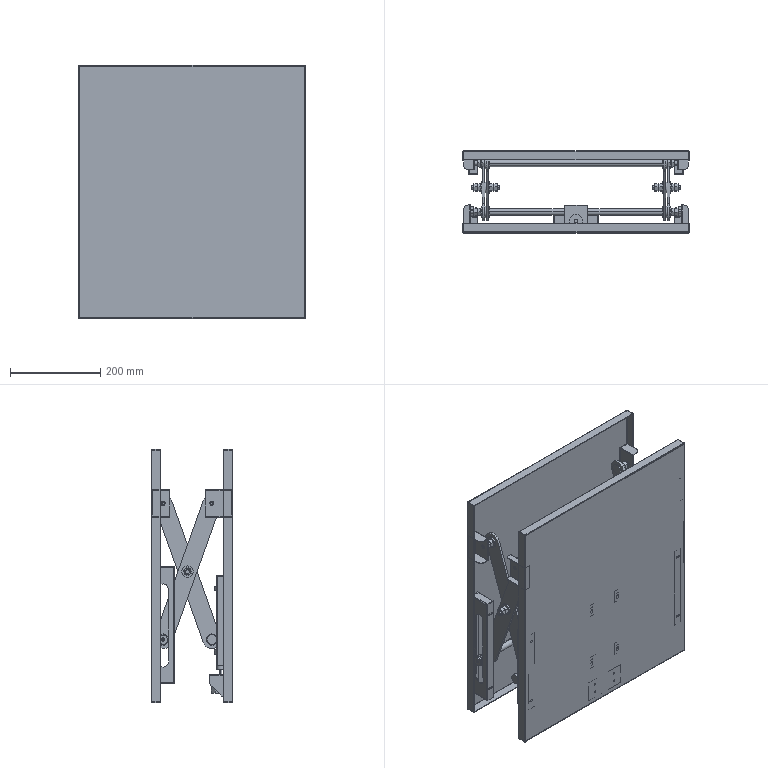Assembly | SolidWorks | mm | 92 component files | 92 solids | 1755 faces | box 500 x 180.82 x 560 mm | volume 1786102 mm3 | plane 890 | cylinder 649 | cone 208 | torus 8 | commonest cylinder face diameters 5 x77 9 x72 0.2 x51 10 x50 19 x48 4 x40 11 x32 25 x32
Bill of materials:
42StepperMotor | 1 |  | Prismatic block, square in plan with chamfered vertical corners (octagonal outline), with a short circular boss and a slender cylindrical shaft rising from the centre of one end face; small holes sit near the corners of the end face.
6800Bearing10-19-5 | 12 |  | Thick annular ring (washer- or spacer-like) with a large central through bore; axial thickness is fairly large compared with the radial wall.
Baffle | 16 |  | Flat annular washer-like disc with a central through hole; thinner than the ring part and with a smaller bore relative to its outer diameter.
Baffle2 | 2 |  | Thin flat disc with a small central through hole (fender-washer-like proportions: large outer diameter relative to the hole).
BearingHousing | 2 |  | Lug or bracket of constant-thickness profile: a rectangular base bar with a rounded (arched) tab rising from its centre. The tab has a through hole on the arch axis, and the base bar has two through holes running perpendicular to the tab hole.
BearingHousingBracket | 2 |  | Sheet-metal hat-section bracket: a central U-shaped channel with an outward flat flange on each side. Each flange has an elongated slot, and the channel web has two small round holes that appear to have slightly raised or formed rims.
AxisFixingPlate | 2 |  | Sheet-metal U/C-channel: a flat rectangular web with two parallel flanges whose free ends are rounded, and a single off-centre round through hole in the web.
BottomPlate | 1 |  | Thin flat rectangular plate, nearly square, with no visible holes or cutouts.
ConnectingRod1 | 4 |  | Thin flat link bar with fully rounded ends and three round through holes: one near each end and one at the midpoint.
Coupling2 | 1 |  | Cylindrical tube or spacer with a concentric through bore; its length is longer than its outer diameter.
FixedRotatingShaft | 4 |  | Flanged, stepped cylindrical pin or bushing: a thin large-diameter disc head, then a short larger-diameter shank section, then a longer slightly smaller-diameter shank. There is an axial bore at the free (small) end.
GuideRail | 2 |  | Elongated sheet-metal folded channel or cover strip of rectangular box-like section. One narrow face has two oblong slots near its ends, and the folded edges show rounded bend corners.
GuideRail2 | 2 |  | Tall, narrow U-shaped channel that looks like bent thin sheet. The web has one long slot that ends in a larger circular opening, like a keyhole. Each side flange has two small slotted holes, one near each end.
hex nuts, style 1-grades ab gb | 24 |  | Hexagonal nut shape with a round hole through the centre and chamfered corners on both faces.
JS60822-7C1L8M6ExternalThreadBearing | 2 |  | Turned stepped pin: a large disc-shaped head, a short collar of middle diameter, and a smaller cylindrical shank.
MotorFixture | 1 |  | Bent bracket that looks like sheet metal, with three faces. The top plate has a large central hole with four small holes in a square around it. One side flange has four holes in a rectangle. The end flange has an angled cut and a rounded corner.
PushRod | 1 |  | Long, slender stepped shaft. The main body is round, and each end steps down twice to a smaller journal. There are two ring-shaped lines near the middle of the body.
PushRod3 | 1 |  | Long, slender stepped shaft like part-63ce, but with a plain main body. Each end steps down twice to smaller diameters.
RotatingShaft | 2 |  | Turned pin with a thin round flange in the middle. A short hub of larger diameter sits on each side of the flange, and a long plain cylindrical section runs out from each hub.
ShaftRetainingRing-15 | 2 |  | Flat, open C-shaped ring with a rectangular cross-section and one gap cut straight through the ring wall.
Slider | 1 |  | Solid rectangular block. The top face has a round through-hole set off-centre, with four smaller holes in a square around it. One end face has a larger round hole set off-centre.
T8LeadScrew | 1 |  | Plain solid cylindrical rod with flat ends.
TLeadScrewNut | 1 |  | Flanged bushing: a round flange with four through-holes, a tube-shaped boss with a central through-bore on one side, and a short spigot on the other side.
AxisFixingPlate2 | 2 |  | U-shaped channel bracket that looks like bent sheet. The back web has one round hole, and the two parallel flanges have one rounded corner each.
TopPlate | 1 |  | Thin flat rectangular plate, close to square (somewhat taller than wide in the face view), with uniform thickness and plain flat faces.
U8-24-11SlotWidth6SlotDepth2 | 2 |  | Round wheel or disc shaped like a pulley, with a central through bore and a concave, rounded (roughly semicircular) groove around its outer edge between two flat-sided flanges.
Mates:
1. coincident | 42StepperMotor-1 face at (0, 0, 0) dir (0, 0, 1) | assembly plane at (0, 0, 0) dir (0, 0, 1)
2. coincident | 42StepperMotor-1 plane at (0, 0, -39) dir (0, 1, 0) | assembly plane at (0, 0, 0) dir (0, 1, 0)
3. coincident | 42StepperMotor-1 plane at (0, 0, -39) dir (1, 0, 0) | assembly plane at (0, 0, 0) dir (1, 0, 0)
4. concentric | 42StepperMotor-1 face at (0, 0, 2) dir (0, 0, -1) r 11 | MotorFixture-1 face at (0, 0, -33.941) dir (0, 0, 1) r 12
5. coincident | 42StepperMotor-1 face at (0, 0, 0) dir (0, 0, 1) | MotorFixture-1 face at (0, -25, 0) dir (0, 0, -1)
6. parallel | 42StepperMotor-1 face at (-21, 21, 0) dir (0, 1, 0) | MotorFixture-1 face at (0, -25, 1.5) dir (0, -1, 0)
7. concentric | 42StepperMotor-1 face at (0, 0, 22.5) dir (0, 0, -1) r 2.5 | Coupling2-1 face at (0, 0, 6.5) dir (0, 0, 1) r 2.5
8. coincident | 42StepperMotor-1 face at (0, 0, 22.5) dir (0, 0, 1) | Coupling2-1 face at (0, 0, 22.5) dir (0, 0, 1)
9. coincident | Coupling2-1 plane at (0, 0, 26) dir (0, -1, 0) | assembly plane at (0, 0, 0) dir (0, 1, 0)
10. concentric | Coupling2-1 face at (0, 0, 22.5) dir (0, 0, 1) r 4 | T8LeadScrew-1 face at (0, 0, 202.5) dir (0, 0, -1) r 4
11. coincident | Coupling2-1 face at (0, 0, 22.5) dir (0, 0, 1) | T8LeadScrew-1 face at (0, 0, 22.5) dir (0, 0, -1)
12. parallel | 42StepperMotor-1 face at (-21, 21, 0) dir (0, 1, 0) | T8LeadScrew-1 plane at (0, 0, 112.5) dir (0, -1, 0)
13. concentric | T8LeadScrew-1 face at (0, 0, 202.5) dir (0, 0, -1) r 4 | BearingHousing-1 face at (0, 0, 56.5) dir (0, 0, -1) r 4
14. parallel | 42StepperMotor-1 face at (-21, 21, 0) dir (0, 1, 0) | BearingHousing-1 face at (14.5, -10, 56.5) dir (0, 1, 0)
15. concentric | T8LeadScrew-1 face at (0, 0, 202.5) dir (0, 0, -1) r 4 | TLeadScrewNut-1 face at (0, 0, 63.712) dir (0, 0, -1) r 4
16. concentric | TLeadScrewNut-1 face at (0, 0, 63.712) dir (0, 0, -1) r 5 | Slider-1 face at (0, 0, 54.787) dir (0, 0, 1) r 5.1
17. coincident | TLeadScrewNut-1 face at (0, 0, 69.212) dir (0, 0, 1) | Slider-1 face at (0, 12.5, 69.212) dir (0, 0, -1)
18. concentric | Slider-1 face at (46.496, 20, 79.212) dir (-1, 0, 0) r 7.6 | PushRod-1 face at (191, 20, 79.212) dir (-1, 0, 0) r 7.5
19. width | PushRod-1 face at (191, 20, 79.212) dir (1, 0, 0) | PushRod-1 face at (-191, 20, 79.212) dir (-1, 0, 0) | Slider-1 face at (-25, 35, 69.212) dir (-1, 0, 0) | Slider-1 face at (25, 35, 69.212) dir (1, 0, 0)
20. parallel | Slider-1 face at (0, 12.5, 69.212) dir (0, 0, -1) | PushRod-1 plane at (0, 20, 79.212) dir (0, 0, 1)
21. concentric | T8LeadScrew-1 face at (0, 0, 202.5) dir (0, 0, -1) r 4 | BearingHousing-2 face at (0, 0, 197.5) dir (0, 0, -1) r 4
22. distance | BearingHousing-2 face at (0, 0, 197.5) dir (0, 0, 1) | T8LeadScrew-1 face at (0, 0, 202.5) dir (0, 0, 1)
23. coincident | BearingHousing-1 face at (14.5, -10, 56.5) dir (0, 1, 0) | BearingHousing-2 face at (14.5, -10, 197.5) dir (0, 1, 0)
24. concentric | PushRod-1 face at (226, 20, 79.212) dir (-1, 0, 0) r 5 | Baffle-1 face at (191, 20, 79.212) dir (1, 0, 0) r 5.5
25. coincident | PushRod-1 face at (191, 20, 79.212) dir (1, 0, 0) | Baffle-1 face at (191, 20, 79.212) dir (-1, 0, 0)
26. concentric | PushRod-1 face at (-226, 20, 79.212) dir (1, 0, 0) r 5 | Baffle-2 face at (-194, 20, 79.212) dir (1, 0, 0) r 5.5
27. coincident | PushRod-1 face at (-191, 20, 79.212) dir (-1, 0, 0) | Baffle-2 face at (-191, 20, 79.212) dir (1, 0, 0)
28. parallel | Baffle-1 plane at (194, 20, 79.212) dir (0, 0, 1) | assembly plane at (0, 0, 0) dir (0, 0, 1)
29. parallel | Baffle-2 plane at (-191, 20, 79.212) dir (0, 0, 1) | assembly plane at (0, 0, 0) dir (0, 0, 1)
30. concentric | PushRod-1 face at (226, 20, 79.212) dir (-1, 0, 0) r 5 | 6800Bearing10-19-5-1 face at (199, 20, 79.212) dir (-1, 0, 0) r 5
31. coincident | Baffle-1 face at (194, 20, 79.212) dir (1, 0, 0) | 6800Bearing10-19-5-1 face at (194, 20, 79.212) dir (-1, 0, 0)
32. parallel | 6800Bearing10-19-5-1 plane at (196.5, 20, 79.212) dir (0, 0, -1) | assembly plane at (0, 0, 0) dir (0, 0, 1)
33. concentric | PushRod-1 face at (-226, 20, 79.212) dir (1, 0, 0) r 5 | 6800Bearing10-19-5-2 face at (-194, 20, 79.212) dir (-1, 0, 0) r 5
34. coincident | Baffle-2 face at (-194, 20, 79.212) dir (-1, 0, 0) | 6800Bearing10-19-5-2 face at (-194, 20, 79.212) dir (1, 0, 0)
35. parallel | 6800Bearing10-19-5-2 plane at (-196.5, 20, 79.212) dir (0, 0, -1) | assembly plane at (0, 0, 0) dir (0, 0, 1)
36. concentric | 6800Bearing10-19-5-1 face at (199, 20, 79.212) dir (-1, 0, 0) r 9.5 | ConnectingRod1-2 face at (225.87, 20, 79.212) dir (-1, 0, 0) r 9.5
37. coincident | Baffle-1 face at (194, 20, 79.212) dir (1, 0, 0) | ConnectingRod1-2 face at (194, 20, 79.212) dir (-1, 0, 0)
38. concentric | 6800Bearing10-19-5-2 face at (-194, 20, 79.212) dir (-1, 0, 0) r 9.5 | ConnectingRod1-3 face at (-167.13, 20, 79.212) dir (-1, 0, 0) r 9.5
39. coincident | Baffle-2 face at (-194, 20, 79.212) dir (-1, 0, 0) | ConnectingRod1-3 face at (-194, 20, 79.212) dir (1, 0, 0)
40. concentric | PushRod-1 face at (226, 20, 79.212) dir (-1, 0, 0) r 5 | Baffle-4 face at (199, 20, 79.212) dir (1, 0, 0) r 5.5
41. coincident | ConnectingRod1-2 face at (199, 20, 79.212) dir (1, 0, 0) | Baffle-4 face at (199, 20, 79.212) dir (-1, 0, 0)
42. concentric | PushRod-1 face at (-226, 20, 79.212) dir (1, 0, 0) r 5 | Baffle-5 face at (-202, 20, 79.212) dir (1, 0, 0) r 5.5
43. coincident | 6800Bearing10-19-5-2 face at (-199, 20, 79.212) dir (-1, 0, 0) | Baffle-5 face at (-199, 20, 79.212) dir (1, 0, 0)
44. parallel | PushRod-1 face at (226, 20, 79.212) dir (1, 0, 0) | Baffle-4 face at (202, 20, 79.212) dir (1, 0, 0)
45. concentric | ConnectingRod1-2 face at (225.87, 73.912, 229.856) dir (-1, 0, 0) r 9.5 | RotatingShaft-1 face at (169, 73.912, 229.856) dir (1, 0, 0) r 5
46. coincident | ConnectingRod1-2 face at (199, 20, 79.212) dir (1, 0, 0) | RotatingShaft-1 face at (199, 73.912, 229.856) dir (-1, 0, 0)
47. concentric | RotatingShaft-1 face at (169, 73.912, 229.856) dir (1, 0, 0) r 5 | 6800Bearing10-19-5-3 face at (199, 73.912, 229.856) dir (-1, 0, 0) r 5
48. coincident | RotatingShaft-1 face at (199, 73.912, 229.856) dir (-1, 0, 0) | 6800Bearing10-19-5-3 face at (199, 73.912, 229.856) dir (1, 0, 0)
49. concentric | RotatingShaft-1 face at (232, 73.912, 229.856) dir (-1, 0, 0) r 5 | 6800Bearing10-19-5-4 face at (207, 73.912, 229.856) dir (-1, 0, 0) r 5
50. coincident | RotatingShaft-1 face at (202, 73.912, 229.856) dir (1, 0, 0) | 6800Bearing10-19-5-4 face at (202, 73.912, 229.856) dir (-1, 0, 0)
51. concentric | 6800Bearing10-19-5-4 face at (207, 73.912, 229.856) dir (-1, 0, 0) r 9.5 | ConnectingRod1-4 face at (175.13, 73.912, 229.856) dir (1, 0, 0) r 9.5
52. coincident | RotatingShaft-1 face at (202, 73.912, 229.856) dir (1, 0, 0) | ConnectingRod1-4 face at (202, 20, 380.5) dir (-1, 0, 0)
53. concentric | ConnectingRod1-3 face at (-167.13, 73.912, 229.856) dir (-1, 0, 0) r 9.5 | RotatingShaft-2 face at (-169, 73.912, 229.856) dir (-1, 0, 0) r 5
54. coincident | ConnectingRod1-3 face at (-199, 20, 79.212) dir (-1, 0, 0) | RotatingShaft-2 face at (-199, 73.912, 229.856) dir (1, 0, 0)
55. concentric | RotatingShaft-1 face at (232, 73.912, 229.856) dir (-1, 0, 0) r 5 | Baffle-6 face at (207, 73.912, 229.856) dir (1, 0, 0) r 5.5
56. coincident | ConnectingRod1-4 face at (207, 20, 380.5) dir (1, 0, 0) | Baffle-6 face at (207, 73.912, 229.856) dir (-1, 0, 0)
57. concentric | RotatingShaft-1 face at (169, 73.912, 229.856) dir (1, 0, 0) r 5 | Baffle-7 face at (191, 73.912, 229.856) dir (1, 0, 0) r 5.5
58. coincident | ConnectingRod1-2 face at (194, 20, 79.212) dir (-1, 0, 0) | Baffle-7 face at (194, 73.912, 229.856) dir (1, 0, 0)
59. concentric | RotatingShaft-2 face at (-169, 73.912, 229.856) dir (-1, 0, 0) r 5 | 6800Bearing10-19-5-5 face at (-194, 73.912, 229.856) dir (-1, 0, 0) r 5
60. coincident | RotatingShaft-2 face at (-199, 73.912, 229.856) dir (1, 0, 0) | 6800Bearing10-19-5-5 face at (-199, 73.912, 229.856) dir (-1, 0, 0)
61. concentric | RotatingShaft-2 face at (-169, 73.912, 229.856) dir (-1, 0, 0) r 5 | Baffle-8 face at (-194, 73.912, 229.856) dir (1, 0, 0) r 5.5
62. coincident | ConnectingRod1-3 face at (-194, 20, 79.212) dir (1, 0, 0) | Baffle-8 face at (-194, 73.912, 229.856) dir (-1, 0, 0)
63. concentric | RotatingShaft-2 face at (-232, 73.912, 229.856) dir (1, 0, 0) r 5 | ConnectingRod1-5 face at (-233.87, 73.912, 229.856) dir (1, 0, 0) r 9.5
64. coincident | RotatingShaft-2 face at (-202, 73.912, 229.856) dir (-1, 0, 0) | ConnectingRod1-5 face at (-202, 20, 380.5) dir (1, 0, 0)
65. concentric | RotatingShaft-2 face at (-232, 73.912, 229.856) dir (1, 0, 0) r 5 | 6800Bearing10-19-5-7 face at (-202, 73.912, 229.856) dir (-1, 0, 0) r 5
66. coincident | RotatingShaft-2 face at (-202, 73.912, 229.856) dir (-1, 0, 0) | 6800Bearing10-19-5-7 face at (-202, 73.912, 229.856) dir (1, 0, 0)
67. concentric | RotatingShaft-2 face at (-232, 73.912, 229.856) dir (1, 0, 0) r 5 | Baffle-9 face at (-210, 73.912, 229.856) dir (1, 0, 0) r 5.5
68. coincident | ConnectingRod1-5 face at (-207, 20, 380.5) dir (-1, 0, 0) | Baffle-9 face at (-207, 73.912, 229.856) dir (1, 0, 0)
69. concentric | ConnectingRod1-3 face at (-167.13, 127.823, 380.5) dir (-1, 0, 0) r 9.5 | 6800Bearing10-19-5-9 face at (-194, 127.823, 380.5) dir (-1, 0, 0) r 5
70. parallel | MotorFixture-1 face at (50, -25, 1.5) dir (1, 0, 0) | Slider-1 face at (25, 35, 69.212) dir (1, 0, 0)
71. concentric | TLeadScrewNut-1 face at (5.657, 5.657, 65.612) dir (0, 0, -1) r 1.7 | Slider-1 face at (5.657, 5.657, 65.677) dir (0, 0, 1) r 1.25
72. concentric | ConnectingRod1-4 face at (175.13, 127.823, 79.212) dir (1, 0, 0) r 9.5 | PushRod3-1 face at (199, 127.823, 79.212) dir (-1, 0, 0) r 7.5
73. concentric | ConnectingRod1-5 face at (-233.87, 127.823, 79.212) dir (1, 0, 0) r 9.5 | PushRod3-1 face at (199, 127.823, 79.212) dir (-1, 0, 0) r 7.5
74. width | ConnectingRod1-5 face at (-202, 20, 380.5) dir (1, 0, 0) | ConnectingRod1-4 face at (202, 20, 380.5) dir (-1, 0, 0) | PushRod3-1 face at (199, 127.823, 79.212) dir (1, 0, 0) | PushRod3-1 face at (-199, 127.823, 79.212) dir (-1, 0, 0)
75. concentric | PushRod3-1 face at (232, 127.823, 79.212) dir (-1, 0, 0) r 5 | Baffle-15 face at (199, 127.823, 79.212) dir (1, 0, 0) r 5.5
76. coincident | PushRod3-1 face at (199, 127.823, 79.212) dir (1, 0, 0) | Baffle-15 face at (199, 127.823, 79.212) dir (-1, 0, 0)
77. concentric | PushRod3-1 face at (-232, 127.823, 79.212) dir (1, 0, 0) r 5 | Baffle-16 face at (-202, 127.823, 79.212) dir (1, 0, 0) r 5.5
78. coincident | PushRod3-1 face at (-199, 127.823, 79.212) dir (-1, 0, 0) | Baffle-16 face at (-199, 127.823, 79.212) dir (1, 0, 0)
79. concentric | PushRod3-1 face at (232, 127.823, 79.212) dir (-1, 0, 0) r 5 | 6800Bearing10-19-5-10 face at (207, 127.823, 79.212) dir (-1, 0, 0) r 5
80. coincident | Baffle-15 face at (202, 127.823, 79.212) dir (1, 0, 0) | 6800Bearing10-19-5-10 face at (202, 127.823, 79.212) dir (-1, 0, 0)
81. coincident | 6800Bearing10-19-5-10 face at (207, 127.823, 79.212) dir (1, 0, 0) | Baffle-17 face at (207, 127.823, 79.212) dir (-1, 0, 0)
82. concentric | PushRod3-1 face at (232, 127.823, 79.212) dir (-1, 0, 0) r 5 | Baffle-17 face at (207, 127.823, 79.212) dir (1, 0, 0) r 5.5
83. concentric | PushRod3-1 face at (-232, 127.823, 79.212) dir (1, 0, 0) r 5 | 6800Bearing10-19-5-11 face at (-202, 127.823, 79.212) dir (-1, 0, 0) r 5
84. coincident | Baffle-16 face at (-202, 127.823, 79.212) dir (-1, 0, 0) | 6800Bearing10-19-5-11 face at (-202, 127.823, 79.212) dir (1, 0, 0)
85. distance | BearingHousing-1 face at (0, 0, 46.5) dir (0, 0, -1) | MotorFixture-1 face at (0, -25, 1.5) dir (0, 0, 1)
86. coincident | GuideRail-1 face at (237, 7.4, 21.5) dir (0, 0, -1) | GuideRail-2 face at (-236.9, -23.4, 21.5) dir (0, 0, -1)
87. concentric | ConnectingRod1-4 face at (175.13, 20, 380.5) dir (1, 0, 0) r 9.5 | FixedRotatingShaft-1 face at (233, 20, 380.5) dir (-1, 0, 0) r 5
88. coincident | ConnectingRod1-4 face at (202, 20, 380.5) dir (-1, 0, 0) | FixedRotatingShaft-1 face at (202, 20, 380.5) dir (1, 0, 0)
89. concentric | FixedRotatingShaft-1 face at (233, 20, 380.5) dir (-1, 0, 0) r 5 | 6800Bearing10-19-5-12 face at (207, 20, 380.5) dir (-1, 0, 0) r 5
90. coincident | FixedRotatingShaft-1 face at (202, 20, 380.5) dir (1, 0, 0) | 6800Bearing10-19-5-12 face at (202, 20, 380.5) dir (-1, 0, 0)
91. coincident | ConnectingRod1-4 face at (207, 20, 380.5) dir (1, 0, 0) | Baffle-19 face at (207, 20, 380.5) dir (-1, 0, 0)
92. concentric | FixedRotatingShaft-1 face at (233, 20, 380.5) dir (-1, 0, 0) r 5 | Baffle-19 face at (207, 20, 380.5) dir (1, 0, 0) r 5.5
93. concentric | ConnectingRod1-5 face at (-233.87, 20, 380.5) dir (1, 0, 0) r 9.5 | FixedRotatingShaft-2 face at (-233, 20, 380.5) dir (1, 0, 0) r 5
94. coincident | ConnectingRod1-5 face at (-202, 20, 380.5) dir (1, 0, 0) | FixedRotatingShaft-2 face at (-202, 20, 380.5) dir (-1, 0, 0)
95. concentric | FixedRotatingShaft-2 face at (-233, 20, 380.5) dir (1, 0, 0) r 5 | 6800Bearing10-19-5-13 face at (-202, 20, 380.5) dir (-1, 0, 0) r 5
96. coincident | FixedRotatingShaft-2 face at (-202, 20, 380.5) dir (-1, 0, 0) | 6800Bearing10-19-5-13 face at (-202, 20, 380.5) dir (1, 0, 0)
97. coincident | 6800Bearing10-19-5-13 face at (-207, 20, 380.5) dir (-1, 0, 0) | Baffle-20 face at (-207, 20, 380.5) dir (1, 0, 0)
98. concentric | FixedRotatingShaft-2 face at (-233, 20, 380.5) dir (1, 0, 0) r 5 | Baffle-20 face at (-210, 20, 380.5) dir (1, 0, 0) r 5.5
99. concentric | FixedRotatingShaft-1 face at (233, 20, 380.5) dir (-1, 0, 0) r 5 | hex nuts, style 1-grades ab gb-1 face at (210, 20, 380.5) dir (1, 0, 0) r 4.5
100. coincident | Baffle-19 face at (210, 20, 380.5) dir (1, 0, 0) | hex nuts, style 1-grades ab gb-1 face at (210, 20, 371.262) dir (-1, 0, 0)
101. concentric | FixedRotatingShaft-1 face at (233, 20, 380.5) dir (-1, 0, 0) r 5 | hex nuts, style 1-grades ab gb-2 face at (226.8, 20, 380.5) dir (-1, 0, 0) r 523.599
102. coincident | hex nuts, style 1-grades ab gb-1 face at (218.4, 20, 371.262) dir (1, 0, 0) | hex nuts, style 1-grades ab gb-2 face at (218.4, 18.848, 389.665) dir (-1, 0, 0)
103. concentric | FixedRotatingShaft-2 face at (-233, 20, 380.5) dir (1, 0, 0) r 5 | hex nuts, style 1-grades ab gb-3 face at (-218.4, 20, 380.5) dir (1, 0, 0) r 4.5
104. coincident | Baffle-20 face at (-210, 20, 380.5) dir (-1, 0, 0) | hex nuts, style 1-grades ab gb-3 face at (-210, 20, 371.262) dir (1, 0, 0)
105. concentric | FixedRotatingShaft-2 face at (-233, 20, 380.5) dir (1, 0, 0) r 5 | hex nuts, style 1-grades ab gb-4 face at (-218.4, 20, 380.5) dir (-1, 0, 0) r 4.5
106. coincident | hex nuts, style 1-grades ab gb-3 face at (-218.4, 20, 371.262) dir (-1, 0, 0) | hex nuts, style 1-grades ab gb-4 face at (-218.4, 18.848, 389.665) dir (1, 0, 0)
107. concentric | PushRod-1 face at (-226, 20, 79.212) dir (1, 0, 0) r 5 | hex nuts, style 1-grades ab gb-5 face at (-202, 20, 79.212) dir (-1, 0, 0) r 4.5
108. coincident | Baffle-5 face at (-202, 20, 79.212) dir (-1, 0, 0) | hex nuts, style 1-grades ab gb-5 face at (-202, 21.525, 88.323) dir (1, 0, 0)
109. concentric | PushRod-1 face at (-226, 20, 79.212) dir (1, 0, 0) r 5 | hex nuts, style 1-grades ab gb-6 face at (-210.4, 20, 79.212) dir (-1, 0, 0) r 4.5
110. coincident | hex nuts, style 1-grades ab gb-5 face at (-210.4, 21.525, 88.323) dir (-1, 0, 0) | hex nuts, style 1-grades ab gb-6 face at (-210.4, 21.525, 88.323) dir (1, 0, 0)
111. concentric | PushRod-1 face at (226, 20, 79.212) dir (-1, 0, 0) r 5 | hex nuts, style 1-grades ab gb-7 face at (210.4, 20, 79.212) dir (-1, 0, 0) r 4.5
112. coincident | Baffle-4 face at (202, 20, 79.212) dir (1, 0, 0) | hex nuts, style 1-grades ab gb-7 face at (202, 21.525, 88.323) dir (-1, 0, 0)
113. concentric | PushRod-1 face at (226, 20, 79.212) dir (-1, 0, 0) r 5 | hex nuts, style 1-grades ab gb-8 face at (218.8, 20, 79.212) dir (-1, 0, 0) r 4.5
114. coincident | hex nuts, style 1-grades ab gb-7 face at (210.4, 21.525, 88.323) dir (1, 0, 0) | hex nuts, style 1-grades ab gb-8 face at (210.4, 21.525, 88.323) dir (-1, 0, 0)
115. concentric | PushRod-1 face at (214, 20, 79.212) dir (1, 0, 0) r 2.5 | JS60822-7C1L8M6ExternalThreadBearing-1 face at (218, 20, 79.212) dir (1, 0, 0) r 3
116. coincident | PushRod-1 face at (226, 20, 79.212) dir (1, 0, 0) | JS60822-7C1L8M6ExternalThreadBearing-1 face at (226, 20, 79.212) dir (-1, 0, 0)
117. concentric | PushRod-1 face at (-214, 20, 79.212) dir (-1, 0, 0) r 2.5 | JS60822-7C1L8M6ExternalThreadBearing-2 face at (-218, 20, 79.212) dir (-1, 0, 0) r 3
118. coincident | PushRod-1 face at (-226, 20, 79.212) dir (-1, 0, 0) | JS60822-7C1L8M6ExternalThreadBearing-2 face at (-226, 20, 79.212) dir (1, 0, 0)
119. concentric | RotatingShaft-1 face at (232, 73.912, 229.856) dir (-1, 0, 0) r 5 | hex nuts, style 1-grades ab gb-9 face at (218.4, 73.912, 229.856) dir (-1, 0, 0) r 4.5
120. coincident | Baffle-6 face at (210, 73.912, 229.856) dir (1, 0, 0) | hex nuts, style 1-grades ab gb-9 face at (210, 75.436, 238.967) dir (-1, 0, 0)
121. concentric | RotatingShaft-1 face at (232, 73.912, 229.856) dir (-1, 0, 0) r 5 | hex nuts, style 1-grades ab gb-10 face at (226.8, 73.912, 229.856) dir (-1, 0, 0) r 4.5
122. coincident | hex nuts, style 1-grades ab gb-9 face at (218.4, 75.436, 238.967) dir (1, 0, 0) | hex nuts, style 1-grades ab gb-10 face at (218.4, 75.436, 238.967) dir (-1, 0, 0)
123. concentric | RotatingShaft-1 face at (169, 73.912, 229.856) dir (1, 0, 0) r 5 | hex nuts, style 1-grades ab gb-11 face at (191, 73.912, 229.856) dir (-1, 0, 0) r 4.5
124. coincident | Baffle-7 face at (191, 73.912, 229.856) dir (-1, 0, 0) | hex nuts, style 1-grades ab gb-11 face at (191, 75.436, 238.967) dir (1, 0, 0)
125. concentric | RotatingShaft-1 face at (169, 73.912, 229.856) dir (1, 0, 0) r 5 | hex nuts, style 1-grades ab gb-12 face at (182.6, 73.912, 229.856) dir (-1, 0, 0) r 4.5
126. coincident | hex nuts, style 1-grades ab gb-11 face at (182.6, 75.436, 238.967) dir (-1, 0, 0) | hex nuts, style 1-grades ab gb-12 face at (182.6, 75.436, 238.967) dir (1, 0, 0)
127. concentric | RotatingShaft-2 face at (-169, 73.912, 229.856) dir (-1, 0, 0) r 5 | hex nuts, style 1-grades ab gb-13 face at (-182.6, 73.912, 229.856) dir (-1, 0, 0) r 4.5
128. coincident | Baffle-8 face at (-191, 73.912, 229.856) dir (1, 0, 0) | hex nuts, style 1-grades ab gb-13 face at (-191, 75.436, 238.967) dir (-1, 0, 0)
129. concentric | RotatingShaft-2 face at (-169, 73.912, 229.856) dir (-1, 0, 0) r 5 | hex nuts, style 1-grades ab gb-14 face at (-174.2, 73.912, 229.856) dir (-1, 0, 0) r 4.5
130. coincident | hex nuts, style 1-grades ab gb-13 face at (-182.6, 75.436, 238.967) dir (1, 0, 0) | hex nuts, style 1-grades ab gb-14 face at (-182.6, 75.436, 238.967) dir (-1, 0, 0)
131. concentric | RotatingShaft-2 face at (-232, 73.912, 229.856) dir (1, 0, 0) r 5 | hex nuts, style 1-grades ab gb-15 face at (-210, 73.912, 229.856) dir (-1, 0, 0) r 4.5
132. coincident | Baffle-9 face at (-210, 73.912, 229.856) dir (-1, 0, 0) | hex nuts, style 1-grades ab gb-15 face at (-210, 75.436, 238.967) dir (1, 0, 0)
133. concentric | RotatingShaft-2 face at (-232, 73.912, 229.856) dir (1, 0, 0) r 5 | hex nuts, style 1-grades ab gb-16 face at (-218.4, 73.912, 229.856) dir (-1, 0, 0) r 4.5
134. coincident | hex nuts, style 1-grades ab gb-15 face at (-218.4, 75.436, 238.967) dir (-1, 0, 0) | hex nuts, style 1-grades ab gb-16 face at (-218.4, 75.436, 238.967) dir (1, 0, 0)
135. coincident | ConnectingRod1-3 face at (-194, 20, 79.212) dir (1, 0, 0) | 6800Bearing10-19-5-9 face at (-194, 127.823, 380.5) dir (1, 0, 0)
136. coincident | ConnectingRod1-2 face at (194, 20, 79.212) dir (-1, 0, 0) | 6800Bearing10-19-5-8 face at (194, 127.823, 380.5) dir (-1, 0, 0)
137. concentric | 6800Bearing10-19-5-9 face at (-194, 127.823, 380.5) dir (-1, 0, 0) r 5 | FixedRotatingShaft-3 face at (-225, 127.823, 380.5) dir (1, 0, 0) r 5
138. coincident | ConnectingRod1-3 face at (-194, 20, 79.212) dir (1, 0, 0) | FixedRotatingShaft-3 face at (-194, 127.823, 380.5) dir (-1, 0, 0)
139. concentric | FixedRotatingShaft-3 face at (-225, 127.823, 380.5) dir (1, 0, 0) r 5 | Baffle-21 face at (-202, 127.823, 380.5) dir (1, 0, 0) r 5.5
140. coincident | ConnectingRod1-3 face at (-199, 20, 79.212) dir (-1, 0, 0) | Baffle-21 face at (-199, 127.823, 380.5) dir (1, 0, 0)
141. concentric | FixedRotatingShaft-3 face at (-225, 127.823, 380.5) dir (1, 0, 0) r 5 | hex nuts, style 1-grades ab gb-18 face at (-210.4, 127.823, 380.5) dir (1, 0, 0) r 4.5
142. coincident | Baffle-21 face at (-202, 127.823, 380.5) dir (-1, 0, 0) | hex nuts, style 1-grades ab gb-18 face at (-202, 127.823, 371.262) dir (1, 0, 0)
143. concentric | FixedRotatingShaft-3 face at (-225, 127.823, 380.5) dir (1, 0, 0) r 5 | hex nuts, style 1-grades ab gb-19 face at (-218.8, 127.823, 380.5) dir (1, 0, 0) r 4.5
144. coincident | hex nuts, style 1-grades ab gb-18 face at (-210.4, 127.823, 371.262) dir (-1, 0, 0) | hex nuts, style 1-grades ab gb-19 face at (-210.4, 127.823, 371.262) dir (1, 0, 0)
145. concentric | 6800Bearing10-19-5-8 face at (199, 127.823, 380.5) dir (-1, 0, 0) r 5 | FixedRotatingShaft-4 face at (225, 127.823, 380.5) dir (-1, 0, 0) r 5
146. coincident | ConnectingRod1-2 face at (194, 20, 79.212) dir (-1, 0, 0) | FixedRotatingShaft-4 face at (194, 127.823, 380.5) dir (1, 0, 0)
147. concentric | FixedRotatingShaft-4 face at (225, 127.823, 380.5) dir (-1, 0, 0) r 5 | Baffle-22 face at (199, 127.823, 380.5) dir (1, 0, 0) r 5.5
148. coincident | ConnectingRod1-2 face at (199, 20, 79.212) dir (1, 0, 0) | Baffle-22 face at (199, 127.823, 380.5) dir (-1, 0, 0)
149. concentric | FixedRotatingShaft-4 face at (225, 127.823, 380.5) dir (-1, 0, 0) r 5 | hex nuts, style 1-grades ab gb-20 face at (210.4, 127.823, 380.5) dir (-1, 0, 0) r 4.5
150. coincident | Baffle-22 face at (202, 127.823, 380.5) dir (1, 0, 0) | hex nuts, style 1-grades ab gb-20 face at (202, 129.348, 389.611) dir (-1, 0, 0)
151. concentric | FixedRotatingShaft-4 face at (225, 127.823, 380.5) dir (-1, 0, 0) r 5 | hex nuts, style 1-grades ab gb-21 face at (218.8, 127.823, 380.5) dir (-1, 0, 0) r 4.5
152. coincident | hex nuts, style 1-grades ab gb-20 face at (210.4, 129.348, 389.611) dir (1, 0, 0) | hex nuts, style 1-grades ab gb-21 face at (210.4, 129.348, 389.611) dir (-1, 0, 0)
153. concentric | TopPlateWelding-1/AxisFixingPlate2-2 face at (-237.607, 127.823, 380.5) dir (1, 0, 0) r 3.75 | FixedRotatingShaft-3 face at (-213, 127.823, 380.5) dir (-1, 0, 0) r 2.5
154. concentric | TopPlateWelding-1/AxisFixingPlate2-1 face at (237.607, 127.823, 380.5) dir (-1, 0, 0) r 3.75 | FixedRotatingShaft-4 face at (213, 127.823, 380.5) dir (1, 0, 0) r 2.5
155. concentric | PushRod3-1 face at (-232, 127.823, 79.212) dir (1, 0, 0) r 5 | Baffle-23 face at (-210, 127.823, 79.212) dir (1, 0, 0) r 5.5
156. coincident | ConnectingRod1-5 face at (-207, 20, 380.5) dir (-1, 0, 0) | Baffle-23 face at (-207, 127.823, 79.212) dir (1, 0, 0)
157. concentric | PushRod3-1 face at (-232, 127.823, 79.212) dir (1, 0, 0) r 5 | hex nuts, style 1-grades ab gb-22 face at (-210, 127.823, 79.212) dir (-1, 0, 0) r 4.5
158. coincident | Baffle-23 face at (-210, 127.823, 79.212) dir (-1, 0, 0) | hex nuts, style 1-grades ab gb-22 face at (-210, 129.348, 88.323) dir (1, 0, 0)
159. concentric | PushRod3-1 face at (-232, 127.823, 79.212) dir (1, 0, 0) r 5 | hex nuts, style 1-grades ab gb-23 face at (-218.4, 127.823, 79.212) dir (-1, 0, 0) r 4.5
160. coincident | hex nuts, style 1-grades ab gb-22 face at (-218.4, 129.348, 88.323) dir (-1, 0, 0) | hex nuts, style 1-grades ab gb-23 face at (-218.4, 129.348, 88.323) dir (1, 0, 0)
161. concentric | PushRod3-1 face at (232, 127.823, 79.212) dir (-1, 0, 0) r 5 | hex nuts, style 1-grades ab gb-24 face at (218.4, 127.823, 79.212) dir (-1, 0, 0) r 4.5
162. coincident | Baffle-17 face at (210, 127.823, 79.212) dir (1, 0, 0) | hex nuts, style 1-grades ab gb-24 face at (210, 129.348, 88.323) dir (-1, 0, 0)
163. concentric | PushRod3-1 face at (232, 127.823, 79.212) dir (-1, 0, 0) r 5 | hex nuts, style 1-grades ab gb-25 face at (226.8, 127.823, 79.212) dir (-1, 0, 0) r 4.5
164. coincident | hex nuts, style 1-grades ab gb-24 face at (218.4, 129.348, 88.323) dir (1, 0, 0) | hex nuts, style 1-grades ab gb-25 face at (218.4, 129.348, 88.323) dir (-1, 0, 0)
165. concentric | PushRod3-1 face at (-243.5, 127.823, 79.212) dir (1, 0, 0) r 4 | U8-24-11SlotWidth6SlotDepth2-1 face at (-266.732, 127.823, 79.212) dir (-1, 0, 0) r 4
166. coincident | PushRod3-1 face at (-232, 127.823, 79.212) dir (-1, 0, 0) | U8-24-11SlotWidth6SlotDepth2-1 face at (-232, 139.823, 79.212) dir (1, 0, 0)
167. concentric | PushRod3-1 face at (243.5, 127.823, 79.212) dir (-1, 0, 0) r 4 | U8-24-11SlotWidth6SlotDepth2-2 face at (208.268, 127.823, 79.212) dir (-1, 0, 0) r 4
168. coincident | PushRod3-1 face at (232, 127.823, 79.212) dir (1, 0, 0) | U8-24-11SlotWidth6SlotDepth2-2 face at (232, 139.823, 79.212) dir (-1, 0, 0)
169. coincident | PushRod3-1 face at (-243.5, 127.823, 79.212) dir (-1, 0, 0) | Baffle2-1 face at (-243.5, 127.823, 79.212) dir (1, 0, 0)
170. concentric | PushRod3-1 face at (-231.5, 127.823, 79.212) dir (-1, 0, 0) r 1.65 | Baffle2-1 face at (-245.5, 127.823, 79.212) dir (1, 0, 0) r 2.5
171. concentric | PushRod3-1 face at (231.5, 127.823, 79.212) dir (1, 0, 0) r 1.65 | Baffle2-2 face at (243.5, 127.823, 79.212) dir (1, 0, 0) r 2.5
172. coincident | PushRod3-1 face at (243.5, 127.823, 79.212) dir (1, 0, 0) | Baffle2-2 face at (243.5, 127.823, 79.212) dir (-1, 0, 0)
173. coincident | TopPlateWelding-1/TopPlate-1 face at (0, 152.823, 220) dir (0, -1, 0) | GuideRail2-1 face at (-218.5, 152.823, -18.5) dir (0, 1, 0)
174. distance | GuideRail2-1 face at (-236.4, 104.923, -18.5) dir (0, 0, -1) | TopPlateWelding-1/TopPlate-1 face at (0, 152.823, -58.5) dir (0, 0, 1)
175. width | U8-24-11SlotWidth6SlotDepth2-1 face at (-243, 139.823, 79.212) dir (-1, 0, 0) | U8-24-11SlotWidth6SlotDepth2-1 face at (-232, 139.823, 79.212) dir (1, 0, 0) | GuideRail2-1 face at (-236.5, 152.823, -18.5) dir (1, 0, 0) | GuideRail2-1 face at (-238.5, 152.823, -18.5) dir (-1, 0, 0)
176. coincident | TopPlateWelding-1/TopPlate-1 face at (0, 152.823, 220) dir (0, -1, 0) | GuideRail2-2 face at (238.5, 152.823, -18.5) dir (0, 1, 0)
177. distance | GuideRail2-2 face at (236.5, 150.723, -18.5) dir (0, 0, -1) | TopPlateWelding-1/TopPlate-1 face at (0, 152.823, -58.5) dir (0, 0, 1)
178. width | U8-24-11SlotWidth6SlotDepth2-2 face at (232, 139.823, 79.212) dir (-1, 0, 0) | U8-24-11SlotWidth6SlotDepth2-2 face at (243, 139.823, 79.212) dir (1, 0, 0) | GuideRail2-2 face at (236.5, 102.823, -18.5) dir (-1, 0, 0) | GuideRail2-2 face at (238.5, 102.823, -18.5) dir (1, 0, 0)
179. coincident | MotorFixture-1 face at (0, -25, 1.5) dir (0, -1, 0) | BottomPlateWelding-2/BottomPlate-1 face at (0, -25, 220) dir (0, 1, 0)
180. width | BottomPlateWelding-2/BottomPlate-1 face at (250, -25, 220) dir (1, 0, 0) | BottomPlateWelding-2/BottomPlate-1 face at (-250, -25, 220) dir (-1, 0, 0) | MotorFixture-1 face at (-50, -25, 1.5) dir (-1, 0, 0) | MotorFixture-1 face at (50, -25, 1.5) dir (1, 0, 0)
181. distance | BottomPlateWelding-2/BottomPlate-1 face at (0, -25, -60) dir (0, 0, -1) | MotorFixture-1 face at (50, -5, -48.5) dir (0, 0, -1)
182. concentric | FixedRotatingShaft-1 face at (233, 20, 380.5) dir (-1, 0, 0) r 5 | BottomPlateWelding-2/AxisFixingPlate-1 face at (245.607, 20, 380.5) dir (-1, 0, 0) r 3.75
183. concentric | FixedRotatingShaft-2 face at (-221, 20, 380.5) dir (-1, 0, 0) r 2.5 | BottomPlateWelding-2/AxisFixingPlate-2 face at (-245.607, 20, 380.5) dir (1, 0, 0) r 3.75
184. distance | GuideRail-1 face at (238.5, 9, 21.5) dir (1, 0, 0) | BottomPlateWelding-2/BottomPlate-1 face at (250, -25, 220) dir (1, 0, 0)
185. distance | GuideRail-1 face at (236.9, -23.4, 21.5) dir (0, 0, -1) | BottomPlateWelding-2/BottomPlate-1 face at (0, -25, -60) dir (0, 0, -1)
186. distance | GuideRail-2 face at (-238.5, 9, 221.5) dir (-1, 0, 0) | BottomPlateWelding-2/BottomPlate-1 face at (-250, -25, 220) dir (-1, 0, 0)
187. coincident | GuideRail-2 face at (-238.5, -25, 221.5) dir (0, -1, 0) | BottomPlateWelding-2/BottomPlate-1 face at (0, -25, 220) dir (0, 1, 0)
188. parallel | TopPlateWelding-1/TopPlate-1 face at (0, 154.323, 220) dir (0, 1, 0) | BottomPlateWelding-2/BottomPlate-1 face at (0, -26.5, 220) dir (0, -1, 0)
189. coincident | GuideRail-1 face at (238.5, -25, 21.5) dir (0, -1, 0) | BottomPlateWelding-2/BottomPlate-1 face at (0, -25, 220) dir (0, 1, 0)
190. coincident | BottomPlateWelding-2/BottomPlate-1 face at (0, -25, 220) dir (0, 1, 0) | BearingHousingBracket-1 face at (-30, -25, 207.5) dir (0, -1, 0)
191. width | BearingHousing-2 face at (-27.5, -10, 197.5) dir (-1, 0, 0) | BearingHousing-2 face at (27.5, -10, 197.5) dir (1, 0, 0) | BearingHousingBracket-1 face at (31, -16, 207.5) dir (1, 0, 0) | BearingHousingBracket-1 face at (-31, -16, 207.5) dir (-1, 0, 0)
192. width | BearingHousingBracket-1 face at (0, -16, 207.5) dir (0, 0, 1) | BearingHousingBracket-1 face at (0, -16, 177.5) dir (0, 0, -1) | BearingHousing-2 face at (0, 0, 187.5) dir (0, 0, -1) | BearingHousing-2 face at (0, 0, 197.5) dir (0, 0, 1)
193. coincident | BottomPlateWelding-2/BottomPlate-1 face at (0, -25, 220) dir (0, 1, 0) | BearingHousingBracket-2 face at (30, -25, 66.5) dir (0, -1, 0)
194. width | BearingHousing-1 face at (27.5, -10, 56.5) dir (1, 0, 0) | BearingHousing-1 face at (-27.5, -10, 56.5) dir (-1, 0, 0) | BearingHousingBracket-2 face at (-31, -16, 66.5) dir (-1, 0, 0) | BearingHousingBracket-2 face at (31, -16, 66.5) dir (1, 0, 0)
195. width | BearingHousing-1 face at (0, 0, 46.5) dir (0, 0, -1) | BearingHousing-1 face at (0, 0, 56.5) dir (0, 0, 1) | BearingHousingBracket-2 face at (0, -16, 66.5) dir (0, 0, 1) | BearingHousingBracket-2 face at (0, -16, 36.5) dir (0, 0, -1)
196. distance | TopPlateWelding-1/TopPlate-1 face at (0, 154.323, 220) dir (0, 1, 0) | BottomPlateWelding-2/BottomPlate-1 face at (0, -26.5, 220) dir (0, -1, 0)
197. concentric | PushRod-1 face at (-26.2, 20, 79.212) dir (1, 0, 0) r 6.5 | ShaftRetainingRing-15-1 face at (-25, 20, 79.212) dir (-1, 0, 0) r 6.5
198. coincident | PushRod-1 face at (-25, 20, 79.212) dir (-1, 0, 0) | ShaftRetainingRing-15-1 face at (-25, 20, 79.212) dir (1, 0, 0)
199. concentric | PushRod-1 face at (26.2, 20, 79.212) dir (-1, 0, 0) r 6.5 | ShaftRetainingRing-15-2 face at (26, 20, 79.212) dir (-1, 0, 0) r 6.5
200. coincident | PushRod-1 face at (25, 20, 79.212) dir (1, 0, 0) | ShaftRetainingRing-15-2 face at (25, 20, 79.212) dir (-1, 0, 0)
201. coincident | BottomPlate-1 plane at (0, 0, 0) dir (1, 0, 0) | BottomPlateWelding plane at (0, 0, 0) dir (1, 0, 0)
202. coincident | BottomPlate-1 plane at (0, 0, 0) dir (0, 0, 1) | BottomPlateWelding plane at (0, 0, 0) dir (0, 0, 1)
203. coincident | BottomPlate-1 plane at (0, 0, 0) dir (0, 1, 0) | BottomPlateWelding plane at (0, 0, 0) dir (0, 1, 0)
204. coincident | BottomPlate-1 face at (0, 0, 0) dir (0, 1, 0) | AxisFixingPlate-1 face at (-233.5, 0, -190.5) dir (0, -1, 0)
205. coincident | BottomPlate-1 face at (-248.5, 0, 0) dir (1, 0, 0) | AxisFixingPlate-1 face at (-248.5, 60, -130.5) dir (-1, 0, 0)
206. distance | AxisFixingPlate-1 face at (-233.5, 0, -190.5) dir (0, 0, -1) | BottomPlate-1 face at (0, 0, -280) dir (0, 0, -1)
207. coincident | BottomPlate-1 face at (0, 0, 0) dir (0, 1, 0) | AxisFixingPlate-2 face at (233.5, 0, -130.5) dir (0, -1, 0)
208. distance | AxisFixingPlate-2 face at (233.5, 0, -190.5) dir (0, 0, -1) | BottomPlate-1 face at (0, 0, -280) dir (0, 0, -1)
209. coincident | BottomPlate-1 face at (248.5, 0, 0) dir (-1, 0, 0) | AxisFixingPlate-2 face at (248.5, 60, -190.5) dir (1, 0, 0)
210. coincident | TopPlate-1 plane at (0, 0, 0) dir (0, 0, 1) | TopPlateWelding plane at (0, 0, 0) dir (0, 0, 1)
211. coincident | TopPlate-1 plane at (0, 0, 0) dir (0, 1, 0) | TopPlateWelding plane at (0, 0, 0) dir (0, 1, 0)
212. coincident | TopPlate-1 plane at (0, 0, 0) dir (1, 0, 0) | TopPlateWelding plane at (0, 0, 0) dir (1, 0, 0)
213. coincident | TopPlate-1 face at (0, 0, 0) dir (0, 1, 0) | AxisFixingPlate2-1 face at (225.5, 0, -130.5) dir (0, -1, 0)
214. coincident | TopPlate-1 face at (248.5, 0, 0) dir (-1, 0, 0) | AxisFixingPlate2-1 face at (248.5, 40, -190.5) dir (1, 0, 0)
215. distance | AxisFixingPlate2-1 face at (225.5, 0, -190.5) dir (0, 0, -1) | TopPlate-1 face at (0, 0, -280) dir (0, 0, -1)
216. coincident | TopPlate-1 face at (0, 0, 0) dir (0, 1, 0) | AxisFixingPlate2-2 face at (-225.5, 0, -190.5) dir (0, -1, 0)
217. coincident | TopPlate-1 face at (-248.5, 0, 0) dir (1, 0, 0) | AxisFixingPlate2-2 face at (-248.5, 1.6, -190.5) dir (-1, 0, 0)
218. distance | AxisFixingPlate2-2 face at (-225.5, 0, -190.5) dir (0, 0, -1) | TopPlate-1 face at (0, 0, -280) dir (0, 0, -1)